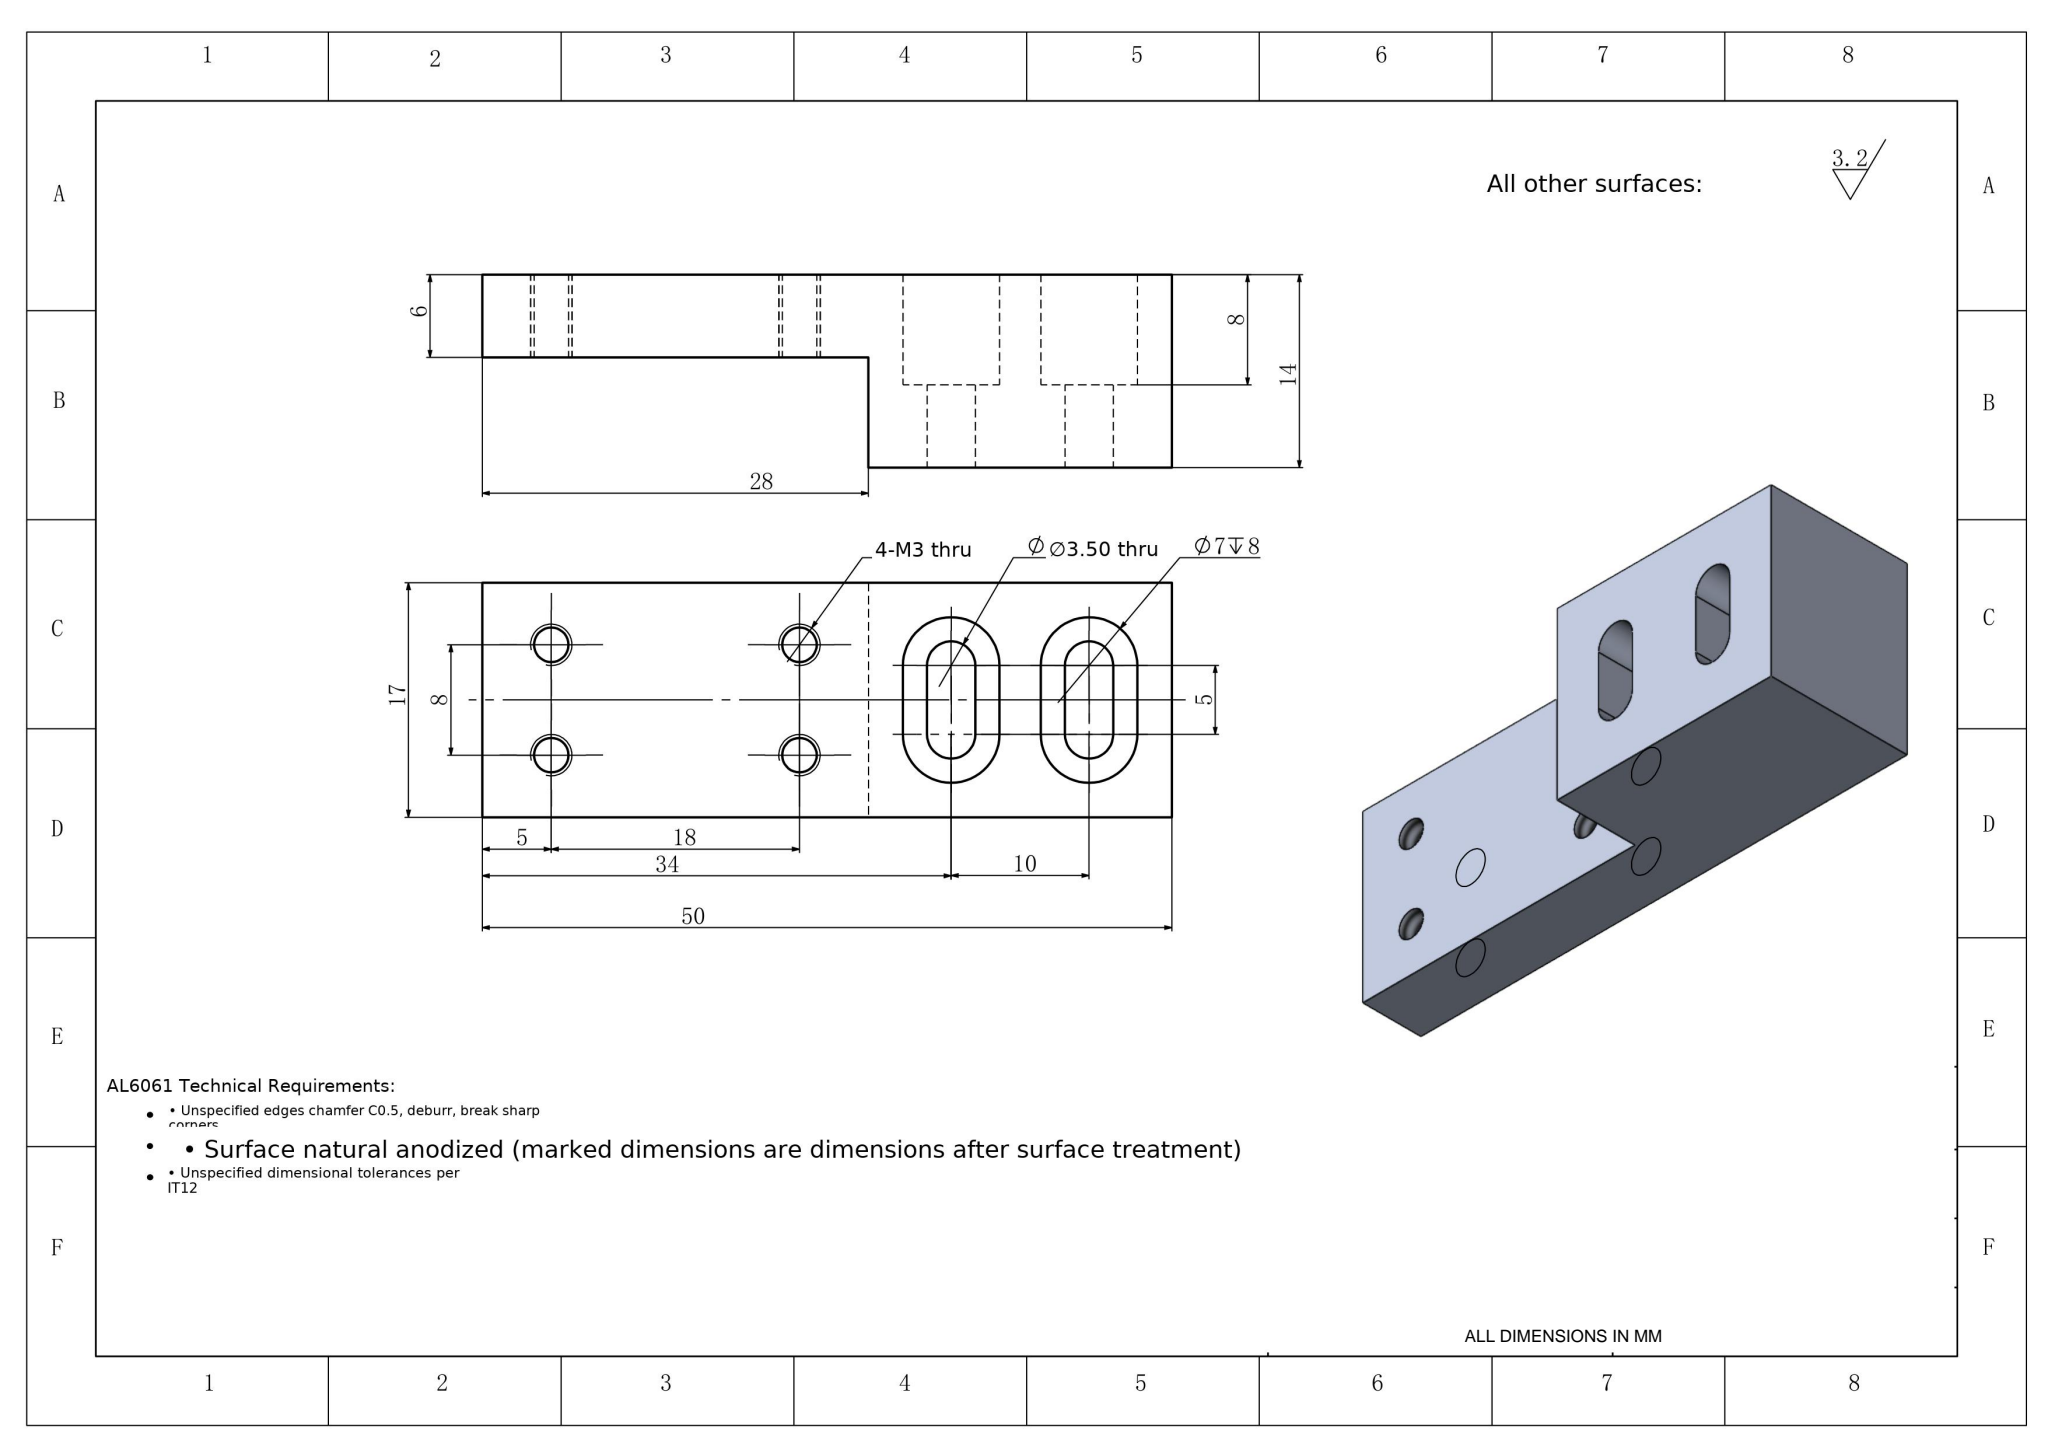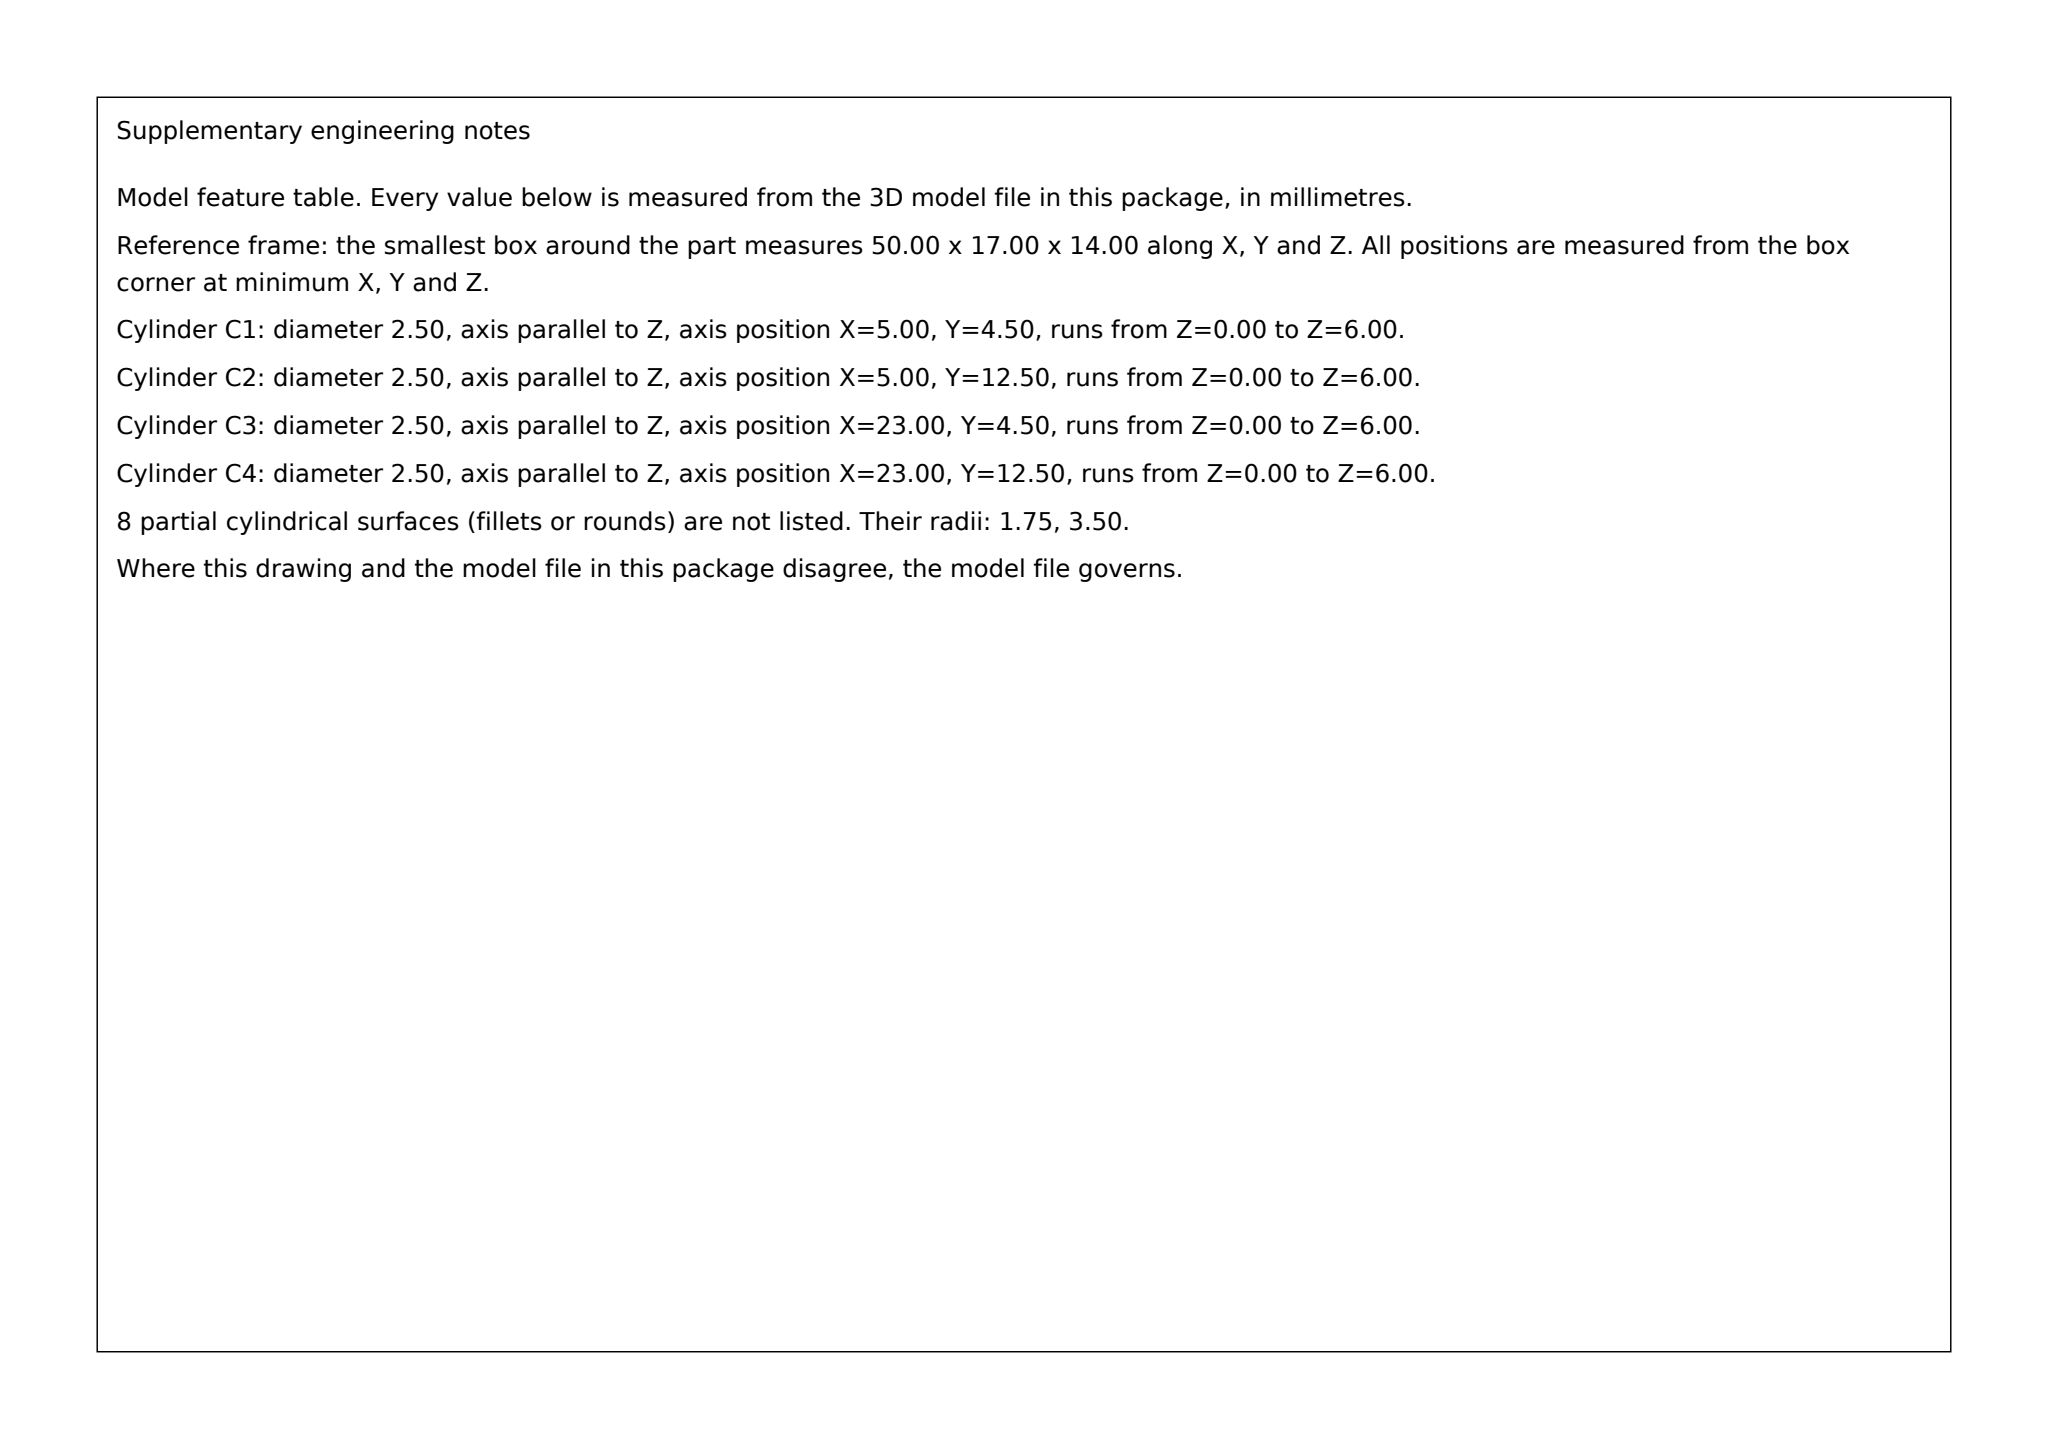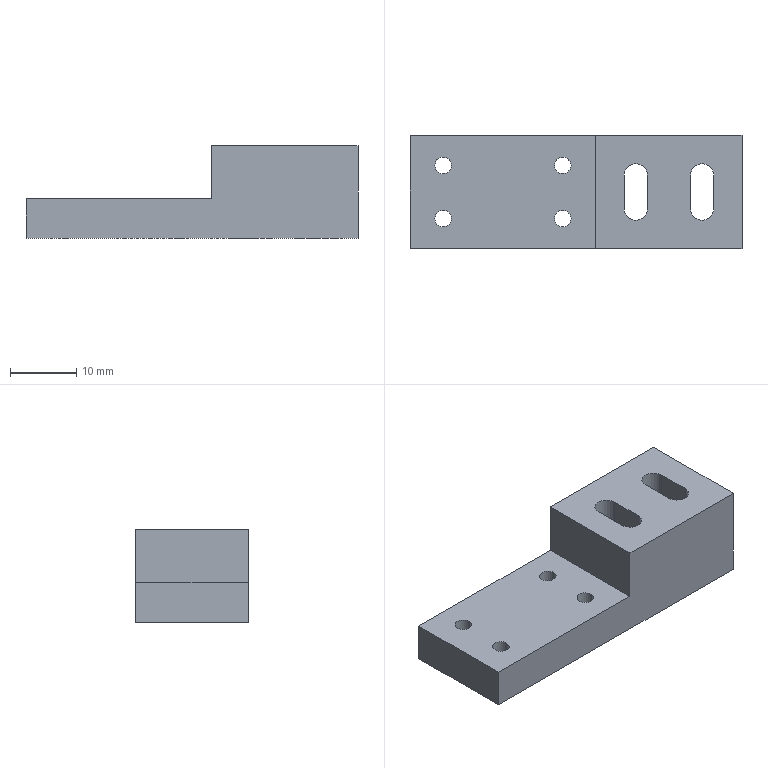Part | SolidWorks | mm | material AL6061 | 1 solid | 34 faces | box 50 x 17 x 14 mm | volume 6473 mm3 | plane 18 | cylinder 16 | commonest cylinder face diameters 2.5 x8 3.5 x4 7 x4
build123d program:
from build123d import *

# Parameters (mm, degrees)
SKETCH1_W           = 50
SKETCH1_H           = 17
BOSS_EXTRUDE1_DEPTH = 14
SKETCH2_W           = 28
SKETCH2_H           = 8
CUT_EXTRUDE1_DEPTH  = 34.317
CUT_EXTRUDE2_DEPTH  = 30.887
CUT_EXTRUDE3_DEPTH  = 8
M3_TAPPED_HOLE1_D   = 2.5


with BuildPart() as part:
    # Sketch1 → Boss-Extrude1 (new body)
    with BuildSketch(Plane.XY):
        Rectangle(SKETCH1_W, SKETCH1_H)
    extrude(amount=BOSS_EXTRUDE1_DEPTH)

    # Sketch2 → Cut-Extrude1 (cut, through all)
    with BuildSketch(Plane(origin=(0, 8.5, 0), x_dir=(1, 0, 0), z_dir=(0, 1, 0))):
        with Locations((-11, -10)):
            Rectangle(SKETCH2_W, SKETCH2_H)
    extrude(amount=-CUT_EXTRUDE1_DEPTH, mode=Mode.SUBTRACT)

    # Sketch3 → Cut-Extrude2 (cut, through all)
    with BuildSketch(Plane(origin=(0, 0, 0), x_dir=(-1, 0, 0), z_dir=(0, 0, -1))):
        with BuildLine():
            Line((-10.75, -2.5), (-10.75, 2.5))
            ThreePointArc((-10.75, 2.5), (-9, 4.25), (-7.25, 2.5))
            Line((-7.25, 2.5), (-7.25, -2.5))
            ThreePointArc((-7.25, -2.5), (-9, -4.25), (-10.75, -2.5))
        make_face()
        with BuildLine():
            Line((-20.75, -2.5), (-20.75, 2.5))
            ThreePointArc((-20.75, 2.5), (-19, 4.25), (-17.25, 2.5))
            Line((-17.25, 2.5), (-17.25, -2.5))
            ThreePointArc((-17.25, -2.5), (-19, -4.25), (-20.75, -2.5))
        make_face()
    extrude(amount=-CUT_EXTRUDE2_DEPTH, mode=Mode.SUBTRACT)

    # Sketch4 → Cut-Extrude3 (cut)
    # profile 1 of 2: a face of its own
    with BuildSketch(Plane(origin=(0, 0, 0), x_dir=(-1, 0, 0), z_dir=(0, 0, -1))):
        with BuildLine():
            Line((-5.5, -2.5), (-5.5, 2.5))
            ThreePointArc((-5.5, 2.5), (-9, 6), (-12.5, 2.5))
            Line((-12.5, 2.5), (-12.5, -2.5))
            ThreePointArc((-12.5, -2.5), (-9, -6), (-5.5, -2.5))
        make_face()
        with BuildLine():
            Line((-7.25, -2.5), (-7.25, 2.5))
            ThreePointArc((-7.25, 2.5), (-9, 4.25), (-10.75, 2.5))
            Line((-10.75, 2.5), (-10.75, -2.5))
            ThreePointArc((-10.75, -2.5), (-9, -4.25), (-7.25, -2.5))
        make_face(mode=Mode.SUBTRACT)
    # profile 2 of 2: a face of its own
    with BuildSketch(Plane(origin=(0, 0, 0), x_dir=(-1, 0, 0), z_dir=(0, 0, -1))):
        with BuildLine():
            Line((-15.5, -2.5), (-15.5, 2.5))
            ThreePointArc((-15.5, 2.5), (-19, 6), (-22.5, 2.5))
            Line((-22.5, 2.5), (-22.5, -2.5))
            ThreePointArc((-22.5, -2.5), (-19, -6), (-15.5, -2.5))
        make_face()
        with BuildLine():
            Line((-20.75, 2.5), (-20.75, -2.5))
            ThreePointArc((-20.75, -2.5), (-19, -4.25), (-17.25, -2.5))
            Line((-17.25, -2.5), (-17.25, 2.5))
            ThreePointArc((-17.25, 2.5), (-19, 4.25), (-20.75, 2.5))
        make_face(mode=Mode.SUBTRACT)
    extrude(amount=-CUT_EXTRUDE3_DEPTH, mode=Mode.SUBTRACT)

    # M3 Tapped Hole1 (through all)
    with Locations(Plane(origin=(0, 0, 0), x_dir=(-1, 0, 0), z_dir=(0, 0, -1))):
        with Locations((20, -4), (20, 4), (2, -4), (2, 4)):
            Hole(M3_TAPPED_HOLE1_D / 2)


solid = part.part